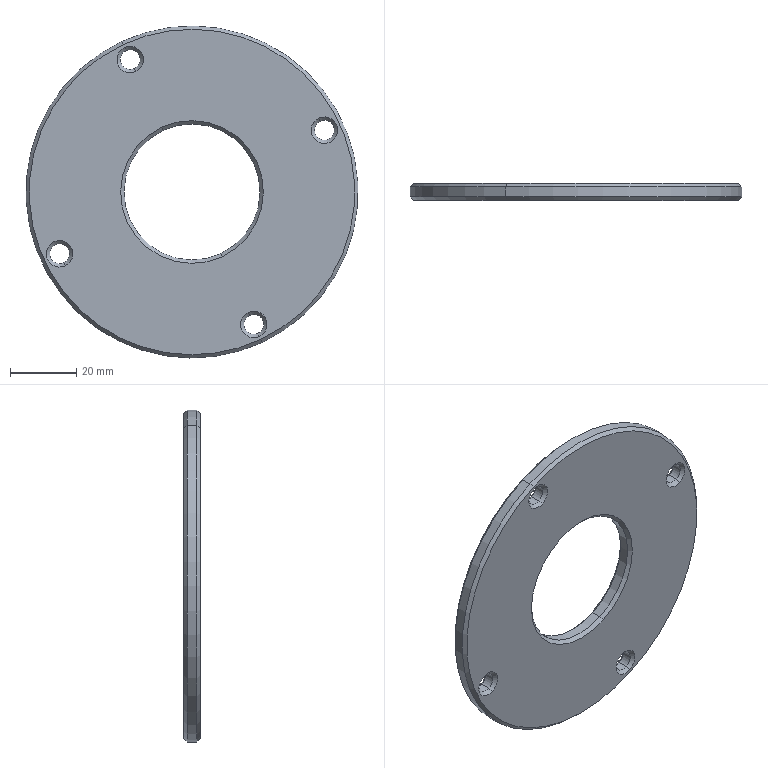Component | SolidWorks | BearingHousingAssembly-1_BearingCoverPlate-1 | 1 solid | 38 faces | box 100 x 5 x 100 mm | volume 31576 mm3 | cone 24 | cylinder 12 | plane 2 | commonest cylinder face diameters 6 x8 41 x2 100 x2 | material Plain Carbon Steel
STEP:
#1=COLOUR_RGB('',0.7922,0.8196,0.9333);
#2=FILL_AREA_STYLE_COLOUR('',#1);
#3=FILL_AREA_STYLE('',(#2));
#4=SURFACE_STYLE_FILL_AREA(#3);
#5=SURFACE_SIDE_STYLE('',(#4));
#6=SURFACE_STYLE_USAGE(.BOTH.,#5);
#7=PRESENTATION_STYLE_ASSIGNMENT((#6));
#8=CARTESIAN_POINT('',(-2.304,9.577,1.441));
#9=VERTEX_POINT('',#8);
#10=CARTESIAN_POINT('',(-2.204,9.577,1.227));
#11=VERTEX_POINT('',#10);
#12=CARTESIAN_POINT('',(-2.254,9.577,1.334));
#13=DIRECTION('',(-0.,-1.,-0.));
#14=DIRECTION('',(0.4226,0.,-0.9063));
#15=AXIS2_PLACEMENT_3D('',#12,#13,#14);
#16=CIRCLE('',#15,0.1181);
#17=EDGE_CURVE('',#9,#11,#16,.T.);
#18=ORIENTED_EDGE('',*,*,#17,.F.);
#19=CARTESIAN_POINT('',(-2.321,9.538,1.476));
#20=VERTEX_POINT('',#19);
#21=CARTESIAN_POINT('',(-2.304,9.577,1.441));
#22=DIRECTION('',(-0.2988,-0.7071,0.6409));
#23=VECTOR('',#22,39.37);
#24=LINE('',#21,#23);
#25=EDGE_CURVE('',#9,#20,#24,.T.);
#26=ORIENTED_EDGE('',*,*,#25,.T.);
#27=CARTESIAN_POINT('',(-2.188,9.538,1.191));
#28=VERTEX_POINT('',#27);
#29=CARTESIAN_POINT('',(-2.254,9.538,1.334));
#30=DIRECTION('',(0.,1.,0.));
#31=DIRECTION('',(0.4226,0.,-0.9063));
#32=AXIS2_PLACEMENT_3D('',#29,#30,#31);
#33=CIRCLE('',#32,0.1575);
#34=EDGE_CURVE('',#28,#20,#33,.T.);
#35=ORIENTED_EDGE('',*,*,#34,.F.);
#36=CARTESIAN_POINT('',(-2.204,9.577,1.227));
#37=DIRECTION('',(0.2988,-0.7071,-0.6409));
#38=VECTOR('',#37,39.37);
#39=LINE('',#36,#38);
#40=EDGE_CURVE('',#11,#28,#39,.T.);
#41=ORIENTED_EDGE('',*,*,#40,.F.);
#42=EDGE_LOOP('',(#18,#26,#35,#41));
#43=FACE_OUTER_BOUND('',#42,.T.);
#44=CARTESIAN_POINT('',(-2.254,9.577,1.334));
#45=DIRECTION('',(-0.,-1.,-0.));
#46=DIRECTION('',(0.4226,0.,-0.9063));
#47=AXIS2_PLACEMENT_3D('',#44,#45,#46);
#48=CONICAL_SURFACE('',#47,0.1181,0.7854);
#49=ADVANCED_FACE('',(#43),#48,.F.);
#50=CARTESIAN_POINT('',(-3.142,9.577,-0.8613));
#51=VERTEX_POINT('',#50);
#52=CARTESIAN_POINT('',(-3.042,9.577,-1.075));
#53=VERTEX_POINT('',#52);
#54=CARTESIAN_POINT('',(-3.092,9.577,-0.9683));
#55=DIRECTION('',(-0.,-1.,-0.));
#56=DIRECTION('',(0.4226,0.,-0.9063));
#57=AXIS2_PLACEMENT_3D('',#54,#55,#56);
#58=CIRCLE('',#57,0.1181);
#59=EDGE_CURVE('',#51,#53,#58,.T.);
#60=ORIENTED_EDGE('',*,*,#59,.F.);
#61=CARTESIAN_POINT('',(-3.159,9.538,-0.8256));
#62=VERTEX_POINT('',#61);
#63=CARTESIAN_POINT('',(-3.142,9.577,-0.8613));
#64=DIRECTION('',(-0.2988,-0.7071,0.6409));
#65=VECTOR('',#64,39.37);
#66=LINE('',#63,#65);
#67=EDGE_CURVE('',#51,#62,#66,.T.);
#68=ORIENTED_EDGE('',*,*,#67,.T.);
#69=CARTESIAN_POINT('',(-3.026,9.538,-1.111));
#70=VERTEX_POINT('',#69);
#71=CARTESIAN_POINT('',(-3.092,9.538,-0.9683));
#72=DIRECTION('',(0.,1.,0.));
#73=DIRECTION('',(0.4226,0.,-0.9063));
#74=AXIS2_PLACEMENT_3D('',#71,#72,#73);
#75=CIRCLE('',#74,0.1575);
#76=EDGE_CURVE('',#70,#62,#75,.T.);
#77=ORIENTED_EDGE('',*,*,#76,.F.);
#78=CARTESIAN_POINT('',(-3.042,9.577,-1.075));
#79=DIRECTION('',(0.2988,-0.7071,-0.6409));
#80=VECTOR('',#79,39.37);
#81=LINE('',#78,#80);
#82=EDGE_CURVE('',#53,#70,#81,.T.);
#83=ORIENTED_EDGE('',*,*,#82,.F.);
#84=EDGE_LOOP('',(#60,#68,#77,#83));
#85=FACE_OUTER_BOUND('',#84,.T.);
#86=CARTESIAN_POINT('',(-3.092,9.577,-0.9683));
#87=DIRECTION('',(-0.,-1.,-0.));
#88=DIRECTION('',(0.4226,0.,-0.9063));
#89=AXIS2_PLACEMENT_3D('',#86,#87,#88);
#90=CONICAL_SURFACE('',#89,0.1181,0.7854);
#91=ADVANCED_FACE('',(#85),#90,.F.);
#92=CARTESIAN_POINT('',(-0.8401,9.577,-1.699));
#93=VERTEX_POINT('',#92);
#94=CARTESIAN_POINT('',(-0.7403,9.577,-1.913));
#95=VERTEX_POINT('',#94);
#96=CARTESIAN_POINT('',(-0.7902,9.577,-1.806));
#97=DIRECTION('',(-0.,-1.,-0.));
#98=DIRECTION('',(0.4226,0.,-0.9063));
#99=AXIS2_PLACEMENT_3D('',#96,#97,#98);
#100=CIRCLE('',#99,0.1181);
#101=EDGE_CURVE('',#93,#95,#100,.T.);
#102=ORIENTED_EDGE('',*,*,#101,.F.);
#103=CARTESIAN_POINT('',(-0.8567,9.538,-1.663));
#104=VERTEX_POINT('',#103);
#105=CARTESIAN_POINT('',(-0.8401,9.577,-1.699));
#106=DIRECTION('',(-0.2988,-0.7071,0.6409));
#107=VECTOR('',#106,39.37);
#108=LINE('',#105,#107);
#109=EDGE_CURVE('',#93,#104,#108,.T.);
#110=ORIENTED_EDGE('',*,*,#109,.T.);
#111=CARTESIAN_POINT('',(-0.7236,9.538,-1.949));
#112=VERTEX_POINT('',#111);
#113=CARTESIAN_POINT('',(-0.7902,9.538,-1.806));
#114=DIRECTION('',(0.,1.,0.));
#115=DIRECTION('',(0.4226,0.,-0.9063));
#116=AXIS2_PLACEMENT_3D('',#113,#114,#115);
#117=CIRCLE('',#116,0.1575);
#118=EDGE_CURVE('',#112,#104,#117,.T.);
#119=ORIENTED_EDGE('',*,*,#118,.F.);
#120=CARTESIAN_POINT('',(-0.7403,9.577,-1.913));
#121=DIRECTION('',(0.2988,-0.7071,-0.6409));
#122=VECTOR('',#121,39.37);
#123=LINE('',#120,#122);
#124=EDGE_CURVE('',#95,#112,#123,.T.);
#125=ORIENTED_EDGE('',*,*,#124,.F.);
#126=EDGE_LOOP('',(#102,#110,#119,#125));
#127=FACE_OUTER_BOUND('',#126,.T.);
#128=CARTESIAN_POINT('',(-0.7902,9.577,-1.806));
#129=DIRECTION('',(-0.,-1.,-0.));
#130=DIRECTION('',(0.4226,0.,-0.9063));
#131=AXIS2_PLACEMENT_3D('',#128,#129,#130);
#132=CONICAL_SURFACE('',#131,0.1181,0.7854);
#133=ADVANCED_FACE('',(#127),#132,.F.);
#134=CARTESIAN_POINT('',(-0.002213,9.577,0.6029));
#135=VERTEX_POINT('',#134);
#136=CARTESIAN_POINT('',(0.09762,9.577,0.3888));
#137=VERTEX_POINT('',#136);
#138=CARTESIAN_POINT('',(0.0477,9.577,0.4959));
#139=DIRECTION('',(-0.,-1.,-0.));
#140=DIRECTION('',(0.4226,0.,-0.9063));
#141=AXIS2_PLACEMENT_3D('',#138,#139,#140);
#142=CIRCLE('',#141,0.1181);
#143=EDGE_CURVE('',#135,#137,#142,.T.);
#144=ORIENTED_EDGE('',*,*,#143,.F.);
#145=CARTESIAN_POINT('',(-0.01885,9.538,0.6386));
#146=VERTEX_POINT('',#145);
#147=CARTESIAN_POINT('',(-0.002213,9.577,0.6029));
#148=DIRECTION('',(-0.2988,-0.7071,0.6409));
#149=VECTOR('',#148,39.37);
#150=LINE('',#147,#149);
#151=EDGE_CURVE('',#135,#146,#150,.T.);
#152=ORIENTED_EDGE('',*,*,#151,.T.);
#153=CARTESIAN_POINT('',(0.1143,9.538,0.3531));
#154=VERTEX_POINT('',#153);
#155=CARTESIAN_POINT('',(0.0477,9.538,0.4959));
#156=DIRECTION('',(0.,1.,0.));
#157=DIRECTION('',(0.4226,0.,-0.9063));
#158=AXIS2_PLACEMENT_3D('',#155,#156,#157);
#159=CIRCLE('',#158,0.1575);
#160=EDGE_CURVE('',#154,#146,#159,.T.);
#161=ORIENTED_EDGE('',*,*,#160,.F.);
#162=CARTESIAN_POINT('',(0.09762,9.577,0.3888));
#163=DIRECTION('',(0.2988,-0.7071,-0.6409));
#164=VECTOR('',#163,39.37);
#165=LINE('',#162,#164);
#166=EDGE_CURVE('',#137,#154,#165,.T.);
#167=ORIENTED_EDGE('',*,*,#166,.F.);
#168=EDGE_LOOP('',(#144,#152,#161,#167));
#169=FACE_OUTER_BOUND('',#168,.T.);
#170=CARTESIAN_POINT('',(0.0477,9.577,0.4959));
#171=DIRECTION('',(-0.,-1.,-0.));
#172=DIRECTION('',(0.4226,0.,-0.9063));
#173=AXIS2_PLACEMENT_3D('',#170,#171,#172);
#174=CONICAL_SURFACE('',#173,0.1181,0.7854);
#175=ADVANCED_FACE('',(#169),#174,.F.);
#176=CARTESIAN_POINT('',(-0.707,9.538,-1.985));
#177=VERTEX_POINT('',#176);
#178=CARTESIAN_POINT('',(-2.338,9.538,1.512));
#179=VERTEX_POINT('',#178);
#180=CARTESIAN_POINT('',(-1.522,9.538,-0.2362));
#181=DIRECTION('',(-0.,-1.,-0.));
#182=DIRECTION('',(0.4226,0.,-0.9063));
#183=AXIS2_PLACEMENT_3D('',#180,#181,#182);
#184=CIRCLE('',#183,1.929);
#185=EDGE_CURVE('',#177,#179,#184,.T.);
#186=ORIENTED_EDGE('',*,*,#185,.F.);
#187=CARTESIAN_POINT('',(-0.6904,9.577,-2.02));
#188=VERTEX_POINT('',#187);
#189=CARTESIAN_POINT('',(-0.707,9.538,-1.985));
#190=DIRECTION('',(0.2988,0.7071,-0.6409));
#191=VECTOR('',#190,39.37);
#192=LINE('',#189,#191);
#193=EDGE_CURVE('',#177,#188,#192,.T.);
#194=ORIENTED_EDGE('',*,*,#193,.T.);
#195=CARTESIAN_POINT('',(-2.354,9.577,1.548));
#196=VERTEX_POINT('',#195);
#197=CARTESIAN_POINT('',(-1.522,9.577,-0.2362));
#198=DIRECTION('',(0.,1.,0.));
#199=DIRECTION('',(0.4226,0.,-0.9063));
#200=AXIS2_PLACEMENT_3D('',#197,#198,#199);
#201=CIRCLE('',#200,1.969);
#202=EDGE_CURVE('',#196,#188,#201,.T.);
#203=ORIENTED_EDGE('',*,*,#202,.F.);
#204=CARTESIAN_POINT('',(-2.338,9.538,1.512));
#205=DIRECTION('',(-0.2988,0.7071,0.6409));
#206=VECTOR('',#205,39.37);
#207=LINE('',#204,#206);
#208=EDGE_CURVE('',#179,#196,#207,.T.);
#209=ORIENTED_EDGE('',*,*,#208,.F.);
#210=EDGE_LOOP('',(#186,#194,#203,#209));
#211=FACE_OUTER_BOUND('',#210,.T.);
#212=CARTESIAN_POINT('',(-1.522,9.538,-0.2362));
#213=DIRECTION('',(0.,1.,0.));
#214=DIRECTION('',(-0.4226,0.,0.9063));
#215=AXIS2_PLACEMENT_3D('',#212,#213,#214);
#216=CONICAL_SURFACE('',#215,1.929,0.7854);
#217=ADVANCED_FACE('',(#211),#216,.T.);
#218=CARTESIAN_POINT('',(-1.863,9.577,0.4952));
#219=VERTEX_POINT('',#218);
#220=CARTESIAN_POINT('',(-1.181,9.577,-0.9677));
#221=VERTEX_POINT('',#220);
#222=CARTESIAN_POINT('',(-1.522,9.577,-0.2362));
#223=DIRECTION('',(-0.,-1.,-0.));
#224=DIRECTION('',(0.4226,0.,-0.9063));
#225=AXIS2_PLACEMENT_3D('',#222,#223,#224);
#226=CIRCLE('',#225,0.8071);
#227=EDGE_CURVE('',#219,#221,#226,.T.);
#228=ORIENTED_EDGE('',*,*,#227,.F.);
#229=CARTESIAN_POINT('',(-1.88,9.538,0.5309));
#230=VERTEX_POINT('',#229);
#231=CARTESIAN_POINT('',(-1.863,9.577,0.4952));
#232=DIRECTION('',(-0.2988,-0.7071,0.6409));
#233=VECTOR('',#232,39.37);
#234=LINE('',#231,#233);
#235=EDGE_CURVE('',#219,#230,#234,.T.);
#236=ORIENTED_EDGE('',*,*,#235,.T.);
#237=CARTESIAN_POINT('',(-1.165,9.538,-1.003));
#238=VERTEX_POINT('',#237);
#239=CARTESIAN_POINT('',(-1.522,9.538,-0.2362));
#240=DIRECTION('',(0.,1.,0.));
#241=DIRECTION('',(0.4226,0.,-0.9063));
#242=AXIS2_PLACEMENT_3D('',#239,#240,#241);
#243=CIRCLE('',#242,0.8465);
#244=EDGE_CURVE('',#238,#230,#243,.T.);
#245=ORIENTED_EDGE('',*,*,#244,.F.);
#246=CARTESIAN_POINT('',(-1.181,9.577,-0.9677));
#247=DIRECTION('',(0.2988,-0.7071,-0.6409));
#248=VECTOR('',#247,39.37);
#249=LINE('',#246,#248);
#250=EDGE_CURVE('',#221,#238,#249,.T.);
#251=ORIENTED_EDGE('',*,*,#250,.F.);
#252=EDGE_LOOP('',(#228,#236,#245,#251));
#253=FACE_OUTER_BOUND('',#252,.T.);
#254=CARTESIAN_POINT('',(-1.522,9.577,-0.2362));
#255=DIRECTION('',(-0.,-1.,-0.));
#256=DIRECTION('',(0.4226,0.,-0.9063));
#257=AXIS2_PLACEMENT_3D('',#254,#255,#256);
#258=CONICAL_SURFACE('',#257,0.8071,0.7854);
#259=ADVANCED_FACE('',(#253),#258,.F.);
#260=CARTESIAN_POINT('',(-2.204,9.695,1.227));
#261=VERTEX_POINT('',#260);
#262=CARTESIAN_POINT('',(-2.304,9.695,1.441));
#263=VERTEX_POINT('',#262);
#264=CARTESIAN_POINT('',(-2.254,9.695,1.334));
#265=DIRECTION('',(0.,1.,0.));
#266=DIRECTION('',(0.4226,0.,-0.9063));
#267=AXIS2_PLACEMENT_3D('',#264,#265,#266);
#268=CIRCLE('',#267,0.1181);
#269=EDGE_CURVE('',#261,#263,#268,.T.);
#270=ORIENTED_EDGE('',*,*,#269,.F.);
#271=CARTESIAN_POINT('',(-2.188,9.735,1.191));
#272=VERTEX_POINT('',#271);
#273=CARTESIAN_POINT('',(-2.188,9.735,1.191));
#274=DIRECTION('',(0.2988,0.7071,-0.6409));
#275=VECTOR('',#274,39.37);
#276=LINE('',#273,#275);
#277=EDGE_CURVE('',#261,#272,#276,.T.);
#278=ORIENTED_EDGE('',*,*,#277,.T.);
#279=CARTESIAN_POINT('',(-2.321,9.735,1.476));
#280=VERTEX_POINT('',#279);
#281=CARTESIAN_POINT('',(-2.254,9.735,1.334));
#282=DIRECTION('',(-0.,-1.,-0.));
#283=DIRECTION('',(0.4226,0.,-0.9063));
#284=AXIS2_PLACEMENT_3D('',#281,#282,#283);
#285=CIRCLE('',#284,0.1575);
#286=EDGE_CURVE('',#280,#272,#285,.T.);
#287=ORIENTED_EDGE('',*,*,#286,.F.);
#288=CARTESIAN_POINT('',(-2.321,9.735,1.476));
#289=DIRECTION('',(-0.2988,0.7071,0.6409));
#290=VECTOR('',#289,39.37);
#291=LINE('',#288,#290);
#292=EDGE_CURVE('',#263,#280,#291,.T.);
#293=ORIENTED_EDGE('',*,*,#292,.F.);
#294=EDGE_LOOP('',(#270,#278,#287,#293));
#295=FACE_OUTER_BOUND('',#294,.T.);
#296=CARTESIAN_POINT('',(-2.254,9.735,1.334));
#297=DIRECTION('',(0.,1.,0.));
#298=DIRECTION('',(-0.4226,0.,0.9063));
#299=AXIS2_PLACEMENT_3D('',#296,#297,#298);
#300=CONICAL_SURFACE('',#299,0.1575,0.7854);
#301=ADVANCED_FACE('',(#295),#300,.F.);
#302=CARTESIAN_POINT('',(-3.042,9.695,-1.075));
#303=VERTEX_POINT('',#302);
#304=CARTESIAN_POINT('',(-3.142,9.695,-0.8613));
#305=VERTEX_POINT('',#304);
#306=CARTESIAN_POINT('',(-3.092,9.695,-0.9683));
#307=DIRECTION('',(0.,1.,0.));
#308=DIRECTION('',(0.4226,0.,-0.9063));
#309=AXIS2_PLACEMENT_3D('',#306,#307,#308);
#310=CIRCLE('',#309,0.1181);
#311=EDGE_CURVE('',#303,#305,#310,.T.);
#312=ORIENTED_EDGE('',*,*,#311,.F.);
#313=CARTESIAN_POINT('',(-3.026,9.735,-1.111));
#314=VERTEX_POINT('',#313);
#315=CARTESIAN_POINT('',(-3.026,9.735,-1.111));
#316=DIRECTION('',(0.2988,0.7071,-0.6409));
#317=VECTOR('',#316,39.37);
#318=LINE('',#315,#317);
#319=EDGE_CURVE('',#303,#314,#318,.T.);
#320=ORIENTED_EDGE('',*,*,#319,.T.);
#321=CARTESIAN_POINT('',(-3.159,9.735,-0.8256));
#322=VERTEX_POINT('',#321);
#323=CARTESIAN_POINT('',(-3.092,9.735,-0.9683));
#324=DIRECTION('',(-0.,-1.,-0.));
#325=DIRECTION('',(0.4226,0.,-0.9063));
#326=AXIS2_PLACEMENT_3D('',#323,#324,#325);
#327=CIRCLE('',#326,0.1575);
#328=EDGE_CURVE('',#322,#314,#327,.T.);
#329=ORIENTED_EDGE('',*,*,#328,.F.);
#330=CARTESIAN_POINT('',(-3.159,9.735,-0.8256));
#331=DIRECTION('',(-0.2988,0.7071,0.6409));
#332=VECTOR('',#331,39.37);
#333=LINE('',#330,#332);
#334=EDGE_CURVE('',#305,#322,#333,.T.);
#335=ORIENTED_EDGE('',*,*,#334,.F.);
#336=EDGE_LOOP('',(#312,#320,#329,#335));
#337=FACE_OUTER_BOUND('',#336,.T.);
#338=CARTESIAN_POINT('',(-3.092,9.735,-0.9683));
#339=DIRECTION('',(0.,1.,0.));
#340=DIRECTION('',(-0.4226,0.,0.9063));
#341=AXIS2_PLACEMENT_3D('',#338,#339,#340);
#342=CONICAL_SURFACE('',#341,0.1575,0.7854);
#343=ADVANCED_FACE('',(#337),#342,.F.);
#344=CARTESIAN_POINT('',(-0.7403,9.695,-1.913));
#345=VERTEX_POINT('',#344);
#346=CARTESIAN_POINT('',(-0.8401,9.695,-1.699));
#347=VERTEX_POINT('',#346);
#348=CARTESIAN_POINT('',(-0.7902,9.695,-1.806));
#349=DIRECTION('',(0.,1.,0.));
#350=DIRECTION('',(0.4226,0.,-0.9063));
#351=AXIS2_PLACEMENT_3D('',#348,#349,#350);
#352=CIRCLE('',#351,0.1181);
#353=EDGE_CURVE('',#345,#347,#352,.T.);
#354=ORIENTED_EDGE('',*,*,#353,.F.);
#355=CARTESIAN_POINT('',(-0.7236,9.735,-1.949));
#356=VERTEX_POINT('',#355);
#357=CARTESIAN_POINT('',(-0.7236,9.735,-1.949));
#358=DIRECTION('',(0.2988,0.7071,-0.6409));
#359=VECTOR('',#358,39.37);
#360=LINE('',#357,#359);
#361=EDGE_CURVE('',#345,#356,#360,.T.);
#362=ORIENTED_EDGE('',*,*,#361,.T.);
#363=CARTESIAN_POINT('',(-0.8567,9.735,-1.663));
#364=VERTEX_POINT('',#363);
#365=CARTESIAN_POINT('',(-0.7902,9.735,-1.806));
#366=DIRECTION('',(-0.,-1.,-0.));
#367=DIRECTION('',(0.4226,0.,-0.9063));
#368=AXIS2_PLACEMENT_3D('',#365,#366,#367);
#369=CIRCLE('',#368,0.1575);
#370=EDGE_CURVE('',#364,#356,#369,.T.);
#371=ORIENTED_EDGE('',*,*,#370,.F.);
#372=CARTESIAN_POINT('',(-0.8567,9.735,-1.663));
#373=DIRECTION('',(-0.2988,0.7071,0.6409));
#374=VECTOR('',#373,39.37);
#375=LINE('',#372,#374);
#376=EDGE_CURVE('',#347,#364,#375,.T.);
#377=ORIENTED_EDGE('',*,*,#376,.F.);
#378=EDGE_LOOP('',(#354,#362,#371,#377));
#379=FACE_OUTER_BOUND('',#378,.T.);
#380=CARTESIAN_POINT('',(-0.7902,9.735,-1.806));
#381=DIRECTION('',(0.,1.,0.));
#382=DIRECTION('',(-0.4226,0.,0.9063));
#383=AXIS2_PLACEMENT_3D('',#380,#381,#382);
#384=CONICAL_SURFACE('',#383,0.1575,0.7854);
#385=ADVANCED_FACE('',(#379),#384,.F.);
#386=CARTESIAN_POINT('',(0.09762,9.695,0.3888));
#387=VERTEX_POINT('',#386);
#388=CARTESIAN_POINT('',(-0.002213,9.695,0.6029));
#389=VERTEX_POINT('',#388);
#390=CARTESIAN_POINT('',(0.0477,9.695,0.4959));
#391=DIRECTION('',(0.,1.,0.));
#392=DIRECTION('',(0.4226,0.,-0.9063));
#393=AXIS2_PLACEMENT_3D('',#390,#391,#392);
#394=CIRCLE('',#393,0.1181);
#395=EDGE_CURVE('',#387,#389,#394,.T.);
#396=ORIENTED_EDGE('',*,*,#395,.F.);
#397=CARTESIAN_POINT('',(0.1143,9.735,0.3531));
#398=VERTEX_POINT('',#397);
#399=CARTESIAN_POINT('',(0.1143,9.735,0.3531));
#400=DIRECTION('',(0.2988,0.7071,-0.6409));
#401=VECTOR('',#400,39.37);
#402=LINE('',#399,#401);
#403=EDGE_CURVE('',#387,#398,#402,.T.);
#404=ORIENTED_EDGE('',*,*,#403,.T.);
#405=CARTESIAN_POINT('',(-0.01885,9.735,0.6386));
#406=VERTEX_POINT('',#405);
#407=CARTESIAN_POINT('',(0.0477,9.735,0.4959));
#408=DIRECTION('',(-0.,-1.,-0.));
#409=DIRECTION('',(0.4226,0.,-0.9063));
#410=AXIS2_PLACEMENT_3D('',#407,#408,#409);
#411=CIRCLE('',#410,0.1575);
#412=EDGE_CURVE('',#406,#398,#411,.T.);
#413=ORIENTED_EDGE('',*,*,#412,.F.);
#414=CARTESIAN_POINT('',(-0.01885,9.735,0.6386));
#415=DIRECTION('',(-0.2988,0.7071,0.6409));
#416=VECTOR('',#415,39.37);
#417=LINE('',#414,#416);
#418=EDGE_CURVE('',#389,#406,#417,.T.);
#419=ORIENTED_EDGE('',*,*,#418,.F.);
#420=EDGE_LOOP('',(#396,#404,#413,#419));
#421=FACE_OUTER_BOUND('',#420,.T.);
#422=CARTESIAN_POINT('',(0.0477,9.735,0.4959));
#423=DIRECTION('',(0.,1.,0.));
#424=DIRECTION('',(-0.4226,0.,0.9063));
#425=AXIS2_PLACEMENT_3D('',#422,#423,#424);
#426=CONICAL_SURFACE('',#425,0.1575,0.7854);
#427=ADVANCED_FACE('',(#421),#426,.F.);
#428=CARTESIAN_POINT('',(-2.338,9.735,1.512));
#429=VERTEX_POINT('',#428);
#430=CARTESIAN_POINT('',(-0.707,9.735,-1.985));
#431=VERTEX_POINT('',#430);
#432=CARTESIAN_POINT('',(-1.522,9.735,-0.2362));
#433=DIRECTION('',(0.,1.,0.));
#434=DIRECTION('',(0.4226,0.,-0.9063));
#435=AXIS2_PLACEMENT_3D('',#432,#433,#434);
#436=CIRCLE('',#435,1.929);
#437=EDGE_CURVE('',#429,#431,#436,.T.);
#438=ORIENTED_EDGE('',*,*,#437,.F.);
#439=CARTESIAN_POINT('',(-2.354,9.695,1.548));
#440=VERTEX_POINT('',#439);
#441=CARTESIAN_POINT('',(-2.354,9.695,1.548));
#442=DIRECTION('',(-0.2988,-0.7071,0.6409));
#443=VECTOR('',#442,39.37);
#444=LINE('',#441,#443);
#445=EDGE_CURVE('',#429,#440,#444,.T.);
#446=ORIENTED_EDGE('',*,*,#445,.T.);
#447=CARTESIAN_POINT('',(-0.6904,9.695,-2.02));
#448=VERTEX_POINT('',#447);
#449=CARTESIAN_POINT('',(-1.522,9.695,-0.2362));
#450=DIRECTION('',(-0.,-1.,-0.));
#451=DIRECTION('',(0.4226,0.,-0.9063));
#452=AXIS2_PLACEMENT_3D('',#449,#450,#451);
#453=CIRCLE('',#452,1.969);
#454=EDGE_CURVE('',#448,#440,#453,.T.);
#455=ORIENTED_EDGE('',*,*,#454,.F.);
#456=CARTESIAN_POINT('',(-0.6904,9.695,-2.02));
#457=DIRECTION('',(0.2988,-0.7071,-0.6409));
#458=VECTOR('',#457,39.37);
#459=LINE('',#456,#458);
#460=EDGE_CURVE('',#431,#448,#459,.T.);
#461=ORIENTED_EDGE('',*,*,#460,.F.);
#462=EDGE_LOOP('',(#438,#446,#455,#461));
#463=FACE_OUTER_BOUND('',#462,.T.);
#464=CARTESIAN_POINT('',(-1.522,9.695,-0.2362));
#465=DIRECTION('',(-0.,-1.,-0.));
#466=DIRECTION('',(0.4226,0.,-0.9063));
#467=AXIS2_PLACEMENT_3D('',#464,#465,#466);
#468=CONICAL_SURFACE('',#467,1.969,0.7854);
#469=ADVANCED_FACE('',(#463),#468,.T.);
#470=CARTESIAN_POINT('',(-1.181,9.695,-0.9677));
#471=VERTEX_POINT('',#470);
#472=CARTESIAN_POINT('',(-1.863,9.695,0.4952));
#473=VERTEX_POINT('',#472);
#474=CARTESIAN_POINT('',(-1.522,9.695,-0.2362));
#475=DIRECTION('',(0.,1.,0.));
#476=DIRECTION('',(0.4226,0.,-0.9063));
#477=AXIS2_PLACEMENT_3D('',#474,#475,#476);
#478=CIRCLE('',#477,0.8071);
#479=EDGE_CURVE('',#471,#473,#478,.T.);
#480=ORIENTED_EDGE('',*,*,#479,.F.);
#481=CARTESIAN_POINT('',(-1.165,9.735,-1.003));
#482=VERTEX_POINT('',#481);
#483=CARTESIAN_POINT('',(-1.165,9.735,-1.003));
#484=DIRECTION('',(0.2988,0.7071,-0.6409));
#485=VECTOR('',#484,39.37);
#486=LINE('',#483,#485);
#487=EDGE_CURVE('',#471,#482,#486,.T.);
#488=ORIENTED_EDGE('',*,*,#487,.T.);
#489=CARTESIAN_POINT('',(-1.88,9.735,0.5309));
#490=VERTEX_POINT('',#489);
#491=CARTESIAN_POINT('',(-1.522,9.735,-0.2362));
#492=DIRECTION('',(-0.,-1.,-0.));
#493=DIRECTION('',(0.4226,0.,-0.9063));
#494=AXIS2_PLACEMENT_3D('',#491,#492,#493);
#495=CIRCLE('',#494,0.8465);
#496=EDGE_CURVE('',#490,#482,#495,.T.);
#497=ORIENTED_EDGE('',*,*,#496,.F.);
#498=CARTESIAN_POINT('',(-1.88,9.735,0.5309));
#499=DIRECTION('',(-0.2988,0.7071,0.6409));
#500=VECTOR('',#499,39.37);
#501=LINE('',#498,#500);
#502=EDGE_CURVE('',#473,#490,#501,.T.);
#503=ORIENTED_EDGE('',*,*,#502,.F.);
#504=EDGE_LOOP('',(#480,#488,#497,#503));
#505=FACE_OUTER_BOUND('',#504,.T.);
#506=CARTESIAN_POINT('',(-1.522,9.735,-0.2362));
#507=DIRECTION('',(0.,1.,0.));
#508=DIRECTION('',(-0.4226,0.,0.9063));
#509=AXIS2_PLACEMENT_3D('',#506,#507,#508);
#510=CONICAL_SURFACE('',#509,0.8465,0.7854);
#511=ADVANCED_FACE('',(#505),#510,.F.);
#512=ORIENTED_EDGE('',*,*,#269,.T.);
#513=CARTESIAN_POINT('',(-2.304,9.735,1.441));
#514=DIRECTION('',(-0.,-1.,-0.));
#515=VECTOR('',#514,39.37);
#516=LINE('',#513,#515);
#517=EDGE_CURVE('',#263,#9,#516,.T.);
#518=ORIENTED_EDGE('',*,*,#517,.T.);
#519=ORIENTED_EDGE('',*,*,#17,.T.);
#520=CARTESIAN_POINT('',(-2.204,9.735,1.227));
#521=DIRECTION('',(-0.,-1.,-0.));
#522=VECTOR('',#521,39.37);
#523=LINE('',#520,#522);
#524=EDGE_CURVE('',#261,#11,#523,.T.);
#525=ORIENTED_EDGE('',*,*,#524,.F.);
#526=EDGE_LOOP('',(#512,#518,#519,#525));
#527=FACE_OUTER_BOUND('',#526,.T.);
#528=CARTESIAN_POINT('',(-2.254,9.735,1.334));
#529=DIRECTION('',(-0.,-1.,-0.));
#530=DIRECTION('',(0.4226,0.,-0.9063));
#531=AXIS2_PLACEMENT_3D('',#528,#529,#530);
#532=CYLINDRICAL_SURFACE('',#531,0.1181);
#533=ADVANCED_FACE('',(#527),#532,.F.);
#534=ORIENTED_EDGE('',*,*,#311,.T.);
#535=CARTESIAN_POINT('',(-3.142,9.735,-0.8613));
#536=DIRECTION('',(-0.,-1.,-0.));
#537=VECTOR('',#536,39.37);
#538=LINE('',#535,#537);
#539=EDGE_CURVE('',#305,#51,#538,.T.);
#540=ORIENTED_EDGE('',*,*,#539,.T.);
#541=ORIENTED_EDGE('',*,*,#59,.T.);
#542=CARTESIAN_POINT('',(-3.042,9.735,-1.075));
#543=DIRECTION('',(-0.,-1.,-0.));
#544=VECTOR('',#543,39.37);
#545=LINE('',#542,#544);
#546=EDGE_CURVE('',#303,#53,#545,.T.);
#547=ORIENTED_EDGE('',*,*,#546,.F.);
#548=EDGE_LOOP('',(#534,#540,#541,#547));
#549=FACE_OUTER_BOUND('',#548,.T.);
#550=CARTESIAN_POINT('',(-3.092,9.735,-0.9683));
#551=DIRECTION('',(-0.,-1.,-0.));
#552=DIRECTION('',(0.4226,0.,-0.9063));
#553=AXIS2_PLACEMENT_3D('',#550,#551,#552);
#554=CYLINDRICAL_SURFACE('',#553,0.1181);
#555=ADVANCED_FACE('',(#549),#554,.F.);
#556=ORIENTED_EDGE('',*,*,#353,.T.);
#557=CARTESIAN_POINT('',(-0.8401,9.735,-1.699));
#558=DIRECTION('',(-0.,-1.,-0.));
#559=VECTOR('',#558,39.37);
#560=LINE('',#557,#559);
#561=EDGE_CURVE('',#347,#93,#560,.T.);
#562=ORIENTED_EDGE('',*,*,#561,.T.);
#563=ORIENTED_EDGE('',*,*,#101,.T.);
#564=CARTESIAN_POINT('',(-0.7403,9.735,-1.913));
#565=DIRECTION('',(-0.,-1.,-0.));
#566=VECTOR('',#565,39.37);
#567=LINE('',#564,#566);
#568=EDGE_CURVE('',#345,#95,#567,.T.);
#569=ORIENTED_EDGE('',*,*,#568,.F.);
#570=EDGE_LOOP('',(#556,#562,#563,#569));
#571=FACE_OUTER_BOUND('',#570,.T.);
#572=CARTESIAN_POINT('',(-0.7902,9.735,-1.806));
#573=DIRECTION('',(-0.,-1.,-0.));
#574=DIRECTION('',(0.4226,0.,-0.9063));
#575=AXIS2_PLACEMENT_3D('',#572,#573,#574);
#576=CYLINDRICAL_SURFACE('',#575,0.1181);
#577=ADVANCED_FACE('',(#571),#576,.F.);
#578=ORIENTED_EDGE('',*,*,#395,.T.);
#579=CARTESIAN_POINT('',(-0.002213,9.735,0.6029));
#580=DIRECTION('',(-0.,-1.,-0.));
#581=VECTOR('',#580,39.37);
#582=LINE('',#579,#581);
#583=EDGE_CURVE('',#389,#135,#582,.T.);
#584=ORIENTED_EDGE('',*,*,#583,.T.);
#585=ORIENTED_EDGE('',*,*,#143,.T.);
#586=CARTESIAN_POINT('',(0.09762,9.735,0.3888));
#587=DIRECTION('',(-0.,-1.,-0.));
#588=VECTOR('',#587,39.37);
#589=LINE('',#586,#588);
#590=EDGE_CURVE('',#387,#137,#589,.T.);
#591=ORIENTED_EDGE('',*,*,#590,.F.);
#592=EDGE_LOOP('',(#578,#584,#585,#591));
#593=FACE_OUTER_BOUND('',#592,.T.);
#594=CARTESIAN_POINT('',(0.0477,9.735,0.4959));
#595=DIRECTION('',(-0.,-1.,-0.));
#596=DIRECTION('',(0.4226,0.,-0.9063));
#597=AXIS2_PLACEMENT_3D('',#594,#595,#596);
#598=CYLINDRICAL_SURFACE('',#597,0.1181);
#599=ADVANCED_FACE('',(#593),#598,.F.);
#600=ORIENTED_EDGE('',*,*,#227,.T.);
#601=CARTESIAN_POINT('',(-1.181,9.538,-0.9677));
#602=DIRECTION('',(0.,1.,0.));
#603=VECTOR('',#602,39.37);
#604=LINE('',#601,#603);
#605=EDGE_CURVE('',#221,#471,#604,.T.);
#606=ORIENTED_EDGE('',*,*,#605,.T.);
#607=ORIENTED_EDGE('',*,*,#479,.T.);
#608=CARTESIAN_POINT('',(-1.863,9.538,0.4952));
#609=DIRECTION('',(0.,1.,0.));
#610=VECTOR('',#609,39.37);
#611=LINE('',#608,#610);
#612=EDGE_CURVE('',#219,#473,#611,.T.);
#613=ORIENTED_EDGE('',*,*,#612,.F.);
#614=EDGE_LOOP('',(#600,#606,#607,#613));
#615=FACE_OUTER_BOUND('',#614,.T.);
#616=CARTESIAN_POINT('',(-1.522,9.538,-0.2362));
#617=DIRECTION('',(0.,1.,0.));
#618=DIRECTION('',(-0.4226,0.,0.9063));
#619=AXIS2_PLACEMENT_3D('',#616,#617,#618);
#620=CYLINDRICAL_SURFACE('',#619,0.8071);
#621=ADVANCED_FACE('',(#615),#620,.F.);
#622=ORIENTED_EDGE('',*,*,#202,.T.);
#623=CARTESIAN_POINT('',(-0.6904,9.538,-2.02));
#624=DIRECTION('',(0.,1.,0.));
#625=VECTOR('',#624,39.37);
#626=LINE('',#623,#625);
#627=EDGE_CURVE('',#188,#448,#626,.T.);
#628=ORIENTED_EDGE('',*,*,#627,.T.);
#629=ORIENTED_EDGE('',*,*,#454,.T.);
#630=CARTESIAN_POINT('',(-2.354,9.538,1.548));
#631=DIRECTION('',(0.,1.,0.));
#632=VECTOR('',#631,39.37);
#633=LINE('',#630,#632);
#634=EDGE_CURVE('',#196,#440,#633,.T.);
#635=ORIENTED_EDGE('',*,*,#634,.F.);
#636=EDGE_LOOP('',(#622,#628,#629,#635));
#637=FACE_OUTER_BOUND('',#636,.T.);
#638=CARTESIAN_POINT('',(-1.522,9.538,-0.2362));
#639=DIRECTION('',(0.,1.,0.));
#640=DIRECTION('',(-0.4226,0.,0.9063));
#641=AXIS2_PLACEMENT_3D('',#638,#639,#640);
#642=CYLINDRICAL_SURFACE('',#641,1.969);
#643=ADVANCED_FACE('',(#637),#642,.T.);
#644=ORIENTED_EDGE('',*,*,#244,.T.);
#645=CARTESIAN_POINT('',(-1.522,9.538,-0.2362));
#646=DIRECTION('',(0.,1.,0.));
#647=DIRECTION('',(0.4226,0.,-0.9063));
#648=AXIS2_PLACEMENT_3D('',#645,#646,#647);
#649=CIRCLE('',#648,0.8465);
#650=EDGE_CURVE('',#230,#238,#649,.T.);
#651=ORIENTED_EDGE('',*,*,#650,.T.);
#652=EDGE_LOOP('',(#644,#651));
#653=FACE_BOUND('',#652,.T.);
#654=CARTESIAN_POINT('',(-1.522,9.538,-0.2362));
#655=DIRECTION('',(-0.,-1.,-0.));
#656=DIRECTION('',(0.4226,0.,-0.9063));
#657=AXIS2_PLACEMENT_3D('',#654,#655,#656);
#658=CIRCLE('',#657,1.929);
#659=EDGE_CURVE('',#179,#177,#658,.T.);
#660=ORIENTED_EDGE('',*,*,#659,.T.);
#661=ORIENTED_EDGE('',*,*,#185,.T.);
#662=EDGE_LOOP('',(#660,#661));
#663=FACE_OUTER_BOUND('',#662,.T.);
#664=ORIENTED_EDGE('',*,*,#160,.T.);
#665=CARTESIAN_POINT('',(0.0477,9.538,0.4959));
#666=DIRECTION('',(0.,1.,0.));
#667=DIRECTION('',(0.4226,0.,-0.9063));
#668=AXIS2_PLACEMENT_3D('',#665,#666,#667);
#669=CIRCLE('',#668,0.1575);
#670=EDGE_CURVE('',#146,#154,#669,.T.);
#671=ORIENTED_EDGE('',*,*,#670,.T.);
#672=EDGE_LOOP('',(#664,#671));
#673=FACE_BOUND('',#672,.T.);
#674=ORIENTED_EDGE('',*,*,#118,.T.);
#675=CARTESIAN_POINT('',(-0.7902,9.538,-1.806));
#676=DIRECTION('',(0.,1.,0.));
#677=DIRECTION('',(0.4226,0.,-0.9063));
#678=AXIS2_PLACEMENT_3D('',#675,#676,#677);
#679=CIRCLE('',#678,0.1575);
#680=EDGE_CURVE('',#104,#112,#679,.T.);
#681=ORIENTED_EDGE('',*,*,#680,.T.);
#682=EDGE_LOOP('',(#674,#681));
#683=FACE_BOUND('',#682,.T.);
#684=ORIENTED_EDGE('',*,*,#76,.T.);
#685=CARTESIAN_POINT('',(-3.092,9.538,-0.9683));
#686=DIRECTION('',(0.,1.,0.));
#687=DIRECTION('',(0.4226,0.,-0.9063));
#688=AXIS2_PLACEMENT_3D('',#685,#686,#687);
#689=CIRCLE('',#688,0.1575);
#690=EDGE_CURVE('',#62,#70,#689,.T.);
#691=ORIENTED_EDGE('',*,*,#690,.T.);
#692=EDGE_LOOP('',(#684,#691));
#693=FACE_BOUND('',#692,.T.);
#694=ORIENTED_EDGE('',*,*,#34,.T.);
#695=CARTESIAN_POINT('',(-2.254,9.538,1.334));
#696=DIRECTION('',(0.,1.,0.));
#697=DIRECTION('',(0.4226,0.,-0.9063));
#698=AXIS2_PLACEMENT_3D('',#695,#696,#697);
#699=CIRCLE('',#698,0.1575);
#700=EDGE_CURVE('',#20,#28,#699,.T.);
#701=ORIENTED_EDGE('',*,*,#700,.T.);
#702=EDGE_LOOP('',(#694,#701));
#703=FACE_BOUND('',#702,.T.);
#704=CARTESIAN_POINT('',(-1.522,9.538,-0.2362));
#705=DIRECTION('',(-0.,-1.,-0.));
#706=DIRECTION('',(0.4226,-0.,-0.9063));
#707=AXIS2_PLACEMENT_3D('',#704,#705,#706);
#708=PLANE('',#707);
#709=ADVANCED_FACE('',(#653,#663,#673,#683,#693,#703),#708,.T.);
#710=ORIENTED_EDGE('',*,*,#496,.T.);
#711=CARTESIAN_POINT('',(-1.522,9.735,-0.2362));
#712=DIRECTION('',(-0.,-1.,-0.));
#713=DIRECTION('',(0.4226,0.,-0.9063));
#714=AXIS2_PLACEMENT_3D('',#711,#712,#713);
#715=CIRCLE('',#714,0.8465);
#716=EDGE_CURVE('',#482,#490,#715,.T.);
#717=ORIENTED_EDGE('',*,*,#716,.T.);
#718=EDGE_LOOP('',(#710,#717));
#719=FACE_BOUND('',#718,.T.);
#720=CARTESIAN_POINT('',(-1.522,9.735,-0.2362));
#721=DIRECTION('',(0.,1.,0.));
#722=DIRECTION('',(0.4226,0.,-0.9063));
#723=AXIS2_PLACEMENT_3D('',#720,#721,#722);
#724=CIRCLE('',#723,1.929);
#725=EDGE_CURVE('',#431,#429,#724,.T.);
#726=ORIENTED_EDGE('',*,*,#725,.T.);
#727=ORIENTED_EDGE('',*,*,#437,.T.);
#728=EDGE_LOOP('',(#726,#727));
#729=FACE_OUTER_BOUND('',#728,.T.);
#730=ORIENTED_EDGE('',*,*,#412,.T.);
#731=CARTESIAN_POINT('',(0.0477,9.735,0.4959));
#732=DIRECTION('',(-0.,-1.,-0.));
#733=DIRECTION('',(0.4226,0.,-0.9063));
#734=AXIS2_PLACEMENT_3D('',#731,#732,#733);
#735=CIRCLE('',#734,0.1575);
#736=EDGE_CURVE('',#398,#406,#735,.T.);
#737=ORIENTED_EDGE('',*,*,#736,.T.);
#738=EDGE_LOOP('',(#730,#737));
#739=FACE_BOUND('',#738,.T.);
#740=ORIENTED_EDGE('',*,*,#370,.T.);
#741=CARTESIAN_POINT('',(-0.7902,9.735,-1.806));
#742=DIRECTION('',(-0.,-1.,-0.));
#743=DIRECTION('',(0.4226,0.,-0.9063));
#744=AXIS2_PLACEMENT_3D('',#741,#742,#743);
#745=CIRCLE('',#744,0.1575);
#746=EDGE_CURVE('',#356,#364,#745,.T.);
#747=ORIENTED_EDGE('',*,*,#746,.T.);
#748=EDGE_LOOP('',(#740,#747));
#749=FACE_BOUND('',#748,.T.);
#750=ORIENTED_EDGE('',*,*,#328,.T.);
#751=CARTESIAN_POINT('',(-3.092,9.735,-0.9683));
#752=DIRECTION('',(-0.,-1.,-0.));
#753=DIRECTION('',(0.4226,0.,-0.9063));
#754=AXIS2_PLACEMENT_3D('',#751,#752,#753);
#755=CIRCLE('',#754,0.1575);
#756=EDGE_CURVE('',#314,#322,#755,.T.);
#757=ORIENTED_EDGE('',*,*,#756,.T.);
#758=EDGE_LOOP('',(#750,#757));
#759=FACE_BOUND('',#758,.T.);
#760=ORIENTED_EDGE('',*,*,#286,.T.);
#761=CARTESIAN_POINT('',(-2.254,9.735,1.334));
#762=DIRECTION('',(-0.,-1.,-0.));
#763=DIRECTION('',(0.4226,0.,-0.9063));
#764=AXIS2_PLACEMENT_3D('',#761,#762,#763);
#765=CIRCLE('',#764,0.1575);
#766=EDGE_CURVE('',#272,#280,#765,.T.);
#767=ORIENTED_EDGE('',*,*,#766,.T.);
#768=EDGE_LOOP('',(#760,#767));
#769=FACE_BOUND('',#768,.T.);
#770=CARTESIAN_POINT('',(-1.522,9.735,-0.2362));
#771=DIRECTION('',(-0.,-1.,-0.));
#772=DIRECTION('',(0.4226,-0.,-0.9063));
#773=AXIS2_PLACEMENT_3D('',#770,#771,#772);
#774=PLANE('',#773);
#775=ADVANCED_FACE('',(#719,#729,#739,#749,#759,#769),#774,.F.);
#776=ORIENTED_EDGE('',*,*,#627,.F.);
#777=CARTESIAN_POINT('',(-1.522,9.577,-0.2362));
#778=DIRECTION('',(0.,1.,0.));
#779=DIRECTION('',(0.4226,0.,-0.9063));
#780=AXIS2_PLACEMENT_3D('',#777,#778,#779);
#781=CIRCLE('',#780,1.969);
#782=EDGE_CURVE('',#188,#196,#781,.T.);
#783=ORIENTED_EDGE('',*,*,#782,.T.);
#784=ORIENTED_EDGE('',*,*,#634,.T.);
#785=CARTESIAN_POINT('',(-1.522,9.695,-0.2362));
#786=DIRECTION('',(-0.,-1.,-0.));
#787=DIRECTION('',(0.4226,0.,-0.9063));
#788=AXIS2_PLACEMENT_3D('',#785,#786,#787);
#789=CIRCLE('',#788,1.969);
#790=EDGE_CURVE('',#440,#448,#789,.T.);
#791=ORIENTED_EDGE('',*,*,#790,.T.);
#792=EDGE_LOOP('',(#776,#783,#784,#791));
#793=FACE_OUTER_BOUND('',#792,.T.);
#794=CARTESIAN_POINT('',(-1.522,9.538,-0.2362));
#795=DIRECTION('',(0.,1.,0.));
#796=DIRECTION('',(-0.4226,0.,0.9063));
#797=AXIS2_PLACEMENT_3D('',#794,#795,#796);
#798=CYLINDRICAL_SURFACE('',#797,1.969);
#799=ADVANCED_FACE('',(#793),#798,.T.);
#800=ORIENTED_EDGE('',*,*,#605,.F.);
#801=CARTESIAN_POINT('',(-1.522,9.577,-0.2362));
#802=DIRECTION('',(-0.,-1.,-0.));
#803=DIRECTION('',(0.4226,0.,-0.9063));
#804=AXIS2_PLACEMENT_3D('',#801,#802,#803);
#805=CIRCLE('',#804,0.8071);
#806=EDGE_CURVE('',#221,#219,#805,.T.);
#807=ORIENTED_EDGE('',*,*,#806,.T.);
#808=ORIENTED_EDGE('',*,*,#612,.T.);
#809=CARTESIAN_POINT('',(-1.522,9.695,-0.2362));
#810=DIRECTION('',(0.,1.,0.));
#811=DIRECTION('',(0.4226,0.,-0.9063));
#812=AXIS2_PLACEMENT_3D('',#809,#810,#811);
#813=CIRCLE('',#812,0.8071);
#814=EDGE_CURVE('',#473,#471,#813,.T.);
#815=ORIENTED_EDGE('',*,*,#814,.T.);
#816=EDGE_LOOP('',(#800,#807,#808,#815));
#817=FACE_OUTER_BOUND('',#816,.T.);
#818=CARTESIAN_POINT('',(-1.522,9.538,-0.2362));
#819=DIRECTION('',(0.,1.,0.));
#820=DIRECTION('',(-0.4226,0.,0.9063));
#821=AXIS2_PLACEMENT_3D('',#818,#819,#820);
#822=CYLINDRICAL_SURFACE('',#821,0.8071);
#823=ADVANCED_FACE('',(#817),#822,.F.);
#824=ORIENTED_EDGE('',*,*,#583,.F.);
#825=CARTESIAN_POINT('',(0.0477,9.695,0.4959));
#826=DIRECTION('',(0.,1.,0.));
#827=DIRECTION('',(0.4226,0.,-0.9063));
#828=AXIS2_PLACEMENT_3D('',#825,#826,#827);
#829=CIRCLE('',#828,0.1181);
#830=EDGE_CURVE('',#389,#387,#829,.T.);
#831=ORIENTED_EDGE('',*,*,#830,.T.);
#832=ORIENTED_EDGE('',*,*,#590,.T.);
#833=CARTESIAN_POINT('',(0.0477,9.577,0.4959));
#834=DIRECTION('',(-0.,-1.,-0.));
#835=DIRECTION('',(0.4226,0.,-0.9063));
#836=AXIS2_PLACEMENT_3D('',#833,#834,#835);
#837=CIRCLE('',#836,0.1181);
#838=EDGE_CURVE('',#137,#135,#837,.T.);
#839=ORIENTED_EDGE('',*,*,#838,.T.);
#840=EDGE_LOOP('',(#824,#831,#832,#839));
#841=FACE_OUTER_BOUND('',#840,.T.);
#842=CARTESIAN_POINT('',(0.0477,9.735,0.4959));
#843=DIRECTION('',(-0.,-1.,-0.));
#844=DIRECTION('',(0.4226,0.,-0.9063));
#845=AXIS2_PLACEMENT_3D('',#842,#843,#844);
#846=CYLINDRICAL_SURFACE('',#845,0.1181);
#847=ADVANCED_FACE('',(#841),#846,.F.);
#848=ORIENTED_EDGE('',*,*,#561,.F.);
#849=CARTESIAN_POINT('',(-0.7902,9.695,-1.806));
#850=DIRECTION('',(0.,1.,0.));
#851=DIRECTION('',(0.4226,0.,-0.9063));
#852=AXIS2_PLACEMENT_3D('',#849,#850,#851);
#853=CIRCLE('',#852,0.1181);
#854=EDGE_CURVE('',#347,#345,#853,.T.);
#855=ORIENTED_EDGE('',*,*,#854,.T.);
#856=ORIENTED_EDGE('',*,*,#568,.T.);
#857=CARTESIAN_POINT('',(-0.7902,9.577,-1.806));
#858=DIRECTION('',(-0.,-1.,-0.));
#859=DIRECTION('',(0.4226,0.,-0.9063));
#860=AXIS2_PLACEMENT_3D('',#857,#858,#859);
#861=CIRCLE('',#860,0.1181);
#862=EDGE_CURVE('',#95,#93,#861,.T.);
#863=ORIENTED_EDGE('',*,*,#862,.T.);
#864=EDGE_LOOP('',(#848,#855,#856,#863));
#865=FACE_OUTER_BOUND('',#864,.T.);
#866=CARTESIAN_POINT('',(-0.7902,9.735,-1.806));
#867=DIRECTION('',(-0.,-1.,-0.));
#868=DIRECTION('',(0.4226,0.,-0.9063));
#869=AXIS2_PLACEMENT_3D('',#866,#867,#868);
#870=CYLINDRICAL_SURFACE('',#869,0.1181);
#871=ADVANCED_FACE('',(#865),#870,.F.);
#872=ORIENTED_EDGE('',*,*,#539,.F.);
#873=CARTESIAN_POINT('',(-3.092,9.695,-0.9683));
#874=DIRECTION('',(0.,1.,0.));
#875=DIRECTION('',(0.4226,0.,-0.9063));
#876=AXIS2_PLACEMENT_3D('',#873,#874,#875);
#877=CIRCLE('',#876,0.1181);
#878=EDGE_CURVE('',#305,#303,#877,.T.);
#879=ORIENTED_EDGE('',*,*,#878,.T.);
#880=ORIENTED_EDGE('',*,*,#546,.T.);
#881=CARTESIAN_POINT('',(-3.092,9.577,-0.9683));
#882=DIRECTION('',(-0.,-1.,-0.));
#883=DIRECTION('',(0.4226,0.,-0.9063));
#884=AXIS2_PLACEMENT_3D('',#881,#882,#883);
#885=CIRCLE('',#884,0.1181);
#886=EDGE_CURVE('',#53,#51,#885,.T.);
#887=ORIENTED_EDGE('',*,*,#886,.T.);
#888=EDGE_LOOP('',(#872,#879,#880,#887));
#889=FACE_OUTER_BOUND('',#888,.T.);
#890=CARTESIAN_POINT('',(-3.092,9.735,-0.9683));
#891=DIRECTION('',(-0.,-1.,-0.));
#892=DIRECTION('',(0.4226,0.,-0.9063));
#893=AXIS2_PLACEMENT_3D('',#890,#891,#892);
#894=CYLINDRICAL_SURFACE('',#893,0.1181);
#895=ADVANCED_FACE('',(#889),#894,.F.);
#896=ORIENTED_EDGE('',*,*,#517,.F.);
#897=CARTESIAN_POINT('',(-2.254,9.695,1.334));
#898=DIRECTION('',(0.,1.,0.));
#899=DIRECTION('',(0.4226,0.,-0.9063));
#900=AXIS2_PLACEMENT_3D('',#897,#898,#899);
#901=CIRCLE('',#900,0.1181);
#902=EDGE_CURVE('',#263,#261,#901,.T.);
#903=ORIENTED_EDGE('',*,*,#902,.T.);
#904=ORIENTED_EDGE('',*,*,#524,.T.);
#905=CARTESIAN_POINT('',(-2.254,9.577,1.334));
#906=DIRECTION('',(-0.,-1.,-0.));
#907=DIRECTION('',(0.4226,0.,-0.9063));
#908=AXIS2_PLACEMENT_3D('',#905,#906,#907);
#909=CIRCLE('',#908,0.1181);
#910=EDGE_CURVE('',#11,#9,#909,.T.);
#911=ORIENTED_EDGE('',*,*,#910,.T.);
#912=EDGE_LOOP('',(#896,#903,#904,#911));
#913=FACE_OUTER_BOUND('',#912,.T.);
#914=CARTESIAN_POINT('',(-2.254,9.735,1.334));
#915=DIRECTION('',(-0.,-1.,-0.));
#916=DIRECTION('',(0.4226,0.,-0.9063));
#917=AXIS2_PLACEMENT_3D('',#914,#915,#916);
#918=CYLINDRICAL_SURFACE('',#917,0.1181);
#919=ADVANCED_FACE('',(#913),#918,.F.);
#920=ORIENTED_EDGE('',*,*,#487,.F.);
#921=ORIENTED_EDGE('',*,*,#814,.F.);
#922=ORIENTED_EDGE('',*,*,#502,.T.);
#923=ORIENTED_EDGE('',*,*,#716,.F.);
#924=EDGE_LOOP('',(#920,#921,#922,#923));
#925=FACE_OUTER_BOUND('',#924,.T.);
#926=CARTESIAN_POINT('',(-1.522,9.735,-0.2362));
#927=DIRECTION('',(0.,1.,0.));
#928=DIRECTION('',(-0.4226,0.,0.9063));
#929=AXIS2_PLACEMENT_3D('',#926,#927,#928);
#930=CONICAL_SURFACE('',#929,0.8465,0.7854);
#931=ADVANCED_FACE('',(#925),#930,.F.);
#932=ORIENTED_EDGE('',*,*,#445,.F.);
#933=ORIENTED_EDGE('',*,*,#725,.F.);
#934=ORIENTED_EDGE('',*,*,#460,.T.);
#935=ORIENTED_EDGE('',*,*,#790,.F.);
#936=EDGE_LOOP('',(#932,#933,#934,#935));
#937=FACE_OUTER_BOUND('',#936,.T.);
#938=CARTESIAN_POINT('',(-1.522,9.695,-0.2362));
#939=DIRECTION('',(-0.,-1.,-0.));
#940=DIRECTION('',(0.4226,0.,-0.9063));
#941=AXIS2_PLACEMENT_3D('',#938,#939,#940);
#942=CONICAL_SURFACE('',#941,1.969,0.7854);
#943=ADVANCED_FACE('',(#937),#942,.T.);
#944=ORIENTED_EDGE('',*,*,#403,.F.);
#945=ORIENTED_EDGE('',*,*,#830,.F.);
#946=ORIENTED_EDGE('',*,*,#418,.T.);
#947=ORIENTED_EDGE('',*,*,#736,.F.);
#948=EDGE_LOOP('',(#944,#945,#946,#947));
#949=FACE_OUTER_BOUND('',#948,.T.);
#950=CARTESIAN_POINT('',(0.0477,9.735,0.4959));
#951=DIRECTION('',(0.,1.,0.));
#952=DIRECTION('',(-0.4226,0.,0.9063));
#953=AXIS2_PLACEMENT_3D('',#950,#951,#952);
#954=CONICAL_SURFACE('',#953,0.1575,0.7854);
#955=ADVANCED_FACE('',(#949),#954,.F.);
#956=ORIENTED_EDGE('',*,*,#361,.F.);
#957=ORIENTED_EDGE('',*,*,#854,.F.);
#958=ORIENTED_EDGE('',*,*,#376,.T.);
#959=ORIENTED_EDGE('',*,*,#746,.F.);
#960=EDGE_LOOP('',(#956,#957,#958,#959));
#961=FACE_OUTER_BOUND('',#960,.T.);
#962=CARTESIAN_POINT('',(-0.7902,9.735,-1.806));
#963=DIRECTION('',(0.,1.,0.));
#964=DIRECTION('',(-0.4226,0.,0.9063));
#965=AXIS2_PLACEMENT_3D('',#962,#963,#964);
#966=CONICAL_SURFACE('',#965,0.1575,0.7854);
#967=ADVANCED_FACE('',(#961),#966,.F.);
#968=ORIENTED_EDGE('',*,*,#319,.F.);
#969=ORIENTED_EDGE('',*,*,#878,.F.);
#970=ORIENTED_EDGE('',*,*,#334,.T.);
#971=ORIENTED_EDGE('',*,*,#756,.F.);
#972=EDGE_LOOP('',(#968,#969,#970,#971));
#973=FACE_OUTER_BOUND('',#972,.T.);
#974=CARTESIAN_POINT('',(-3.092,9.735,-0.9683));
#975=DIRECTION('',(0.,1.,0.));
#976=DIRECTION('',(-0.4226,0.,0.9063));
#977=AXIS2_PLACEMENT_3D('',#974,#975,#976);
#978=CONICAL_SURFACE('',#977,0.1575,0.7854);
#979=ADVANCED_FACE('',(#973),#978,.F.);
#980=ORIENTED_EDGE('',*,*,#277,.F.);
#981=ORIENTED_EDGE('',*,*,#902,.F.);
#982=ORIENTED_EDGE('',*,*,#292,.T.);
#983=ORIENTED_EDGE('',*,*,#766,.F.);
#984=EDGE_LOOP('',(#980,#981,#982,#983));
#985=FACE_OUTER_BOUND('',#984,.T.);
#986=CARTESIAN_POINT('',(-2.254,9.735,1.334));
#987=DIRECTION('',(0.,1.,0.));
#988=DIRECTION('',(-0.4226,0.,0.9063));
#989=AXIS2_PLACEMENT_3D('',#986,#987,#988);
#990=CONICAL_SURFACE('',#989,0.1575,0.7854);
#991=ADVANCED_FACE('',(#985),#990,.F.);
#992=ORIENTED_EDGE('',*,*,#235,.F.);
#993=ORIENTED_EDGE('',*,*,#806,.F.);
#994=ORIENTED_EDGE('',*,*,#250,.T.);
#995=ORIENTED_EDGE('',*,*,#650,.F.);
#996=EDGE_LOOP('',(#992,#993,#994,#995));
#997=FACE_OUTER_BOUND('',#996,.T.);
#998=CARTESIAN_POINT('',(-1.522,9.577,-0.2362));
#999=DIRECTION('',(-0.,-1.,-0.));
#1000=DIRECTION('',(0.4226,0.,-0.9063));
#1001=AXIS2_PLACEMENT_3D('',#998,#999,#1000);
#1002=CONICAL_SURFACE('',#1001,0.8071,0.7854);
#1003=ADVANCED_FACE('',(#997),#1002,.F.);
#1004=ORIENTED_EDGE('',*,*,#193,.F.);
#1005=ORIENTED_EDGE('',*,*,#659,.F.);
#1006=ORIENTED_EDGE('',*,*,#208,.T.);
#1007=ORIENTED_EDGE('',*,*,#782,.F.);
#1008=EDGE_LOOP('',(#1004,#1005,#1006,#1007));
#1009=FACE_OUTER_BOUND('',#1008,.T.);
#1010=CARTESIAN_POINT('',(-1.522,9.538,-0.2362));
#1011=DIRECTION('',(0.,1.,0.));
#1012=DIRECTION('',(-0.4226,0.,0.9063));
#1013=AXIS2_PLACEMENT_3D('',#1010,#1011,#1012);
#1014=CONICAL_SURFACE('',#1013,1.929,0.7854);
#1015=ADVANCED_FACE('',(#1009),#1014,.T.);
#1016=ORIENTED_EDGE('',*,*,#151,.F.);
#1017=ORIENTED_EDGE('',*,*,#838,.F.);
#1018=ORIENTED_EDGE('',*,*,#166,.T.);
#1019=ORIENTED_EDGE('',*,*,#670,.F.);
#1020=EDGE_LOOP('',(#1016,#1017,#1018,#1019));
#1021=FACE_OUTER_BOUND('',#1020,.T.);
#1022=CARTESIAN_POINT('',(0.0477,9.577,0.4959));
#1023=DIRECTION('',(-0.,-1.,-0.));
#1024=DIRECTION('',(0.4226,0.,-0.9063));
#1025=AXIS2_PLACEMENT_3D('',#1022,#1023,#1024);
#1026=CONICAL_SURFACE('',#1025,0.1181,0.7854);
#1027=ADVANCED_FACE('',(#1021),#1026,.F.);
#1028=ORIENTED_EDGE('',*,*,#109,.F.);
#1029=ORIENTED_EDGE('',*,*,#862,.F.);
#1030=ORIENTED_EDGE('',*,*,#124,.T.);
#1031=ORIENTED_EDGE('',*,*,#680,.F.);
#1032=EDGE_LOOP('',(#1028,#1029,#1030,#1031));
#1033=FACE_OUTER_BOUND('',#1032,.T.);
#1034=CARTESIAN_POINT('',(-0.7902,9.577,-1.806));
#1035=DIRECTION('',(-0.,-1.,-0.));
#1036=DIRECTION('',(0.4226,0.,-0.9063));
#1037=AXIS2_PLACEMENT_3D('',#1034,#1035,#1036);
#1038=CONICAL_SURFACE('',#1037,0.1181,0.7854);
#1039=ADVANCED_FACE('',(#1033),#1038,.F.);
#1040=ORIENTED_EDGE('',*,*,#67,.F.);
#1041=ORIENTED_EDGE('',*,*,#886,.F.);
#1042=ORIENTED_EDGE('',*,*,#82,.T.);
#1043=ORIENTED_EDGE('',*,*,#690,.F.);
#1044=EDGE_LOOP('',(#1040,#1041,#1042,#1043));
#1045=FACE_OUTER_BOUND('',#1044,.T.);
#1046=CARTESIAN_POINT('',(-3.092,9.577,-0.9683));
#1047=DIRECTION('',(-0.,-1.,-0.));
#1048=DIRECTION('',(0.4226,0.,-0.9063));
#1049=AXIS2_PLACEMENT_3D('',#1046,#1047,#1048);
#1050=CONICAL_SURFACE('',#1049,0.1181,0.7854);
#1051=ADVANCED_FACE('',(#1045),#1050,.F.);
#1052=ORIENTED_EDGE('',*,*,#25,.F.);
#1053=ORIENTED_EDGE('',*,*,#910,.F.);
#1054=ORIENTED_EDGE('',*,*,#40,.T.);
#1055=ORIENTED_EDGE('',*,*,#700,.F.);
#1056=EDGE_LOOP('',(#1052,#1053,#1054,#1055));
#1057=FACE_OUTER_BOUND('',#1056,.T.);
#1058=CARTESIAN_POINT('',(-2.254,9.577,1.334));
#1059=DIRECTION('',(-0.,-1.,-0.));
#1060=DIRECTION('',(0.4226,0.,-0.9063));
#1061=AXIS2_PLACEMENT_3D('',#1058,#1059,#1060);
#1062=CONICAL_SURFACE('',#1061,0.1181,0.7854);
#1063=ADVANCED_FACE('',(#1057),#1062,.F.);
#1064=CLOSED_SHELL('',(#49,#91,#133,#175,#217,#259,#301,#343,#385,#427,#469,#511,#533,#555,#577,#599,#621,#643,#709,#775,#799,#823,#847,#871,#895,#919,#931,#943,#955,#967,#979,#991,#1003,#1015,#1027,#1039,#1051,#1063));
#1065=MANIFOLD_SOLID_BREP('',#1064);
#1066=STYLED_ITEM('',(#7),#1065);
#1067=PRESENTATION_LAYER_ASSIGNMENT('','',(#1066));
#1068=(LENGTH_UNIT()NAMED_UNIT(*)SI_UNIT($,.METRE.));
#1069=LENGTH_MEASURE_WITH_UNIT(LENGTH_MEASURE(0.0254),#1068);
#1070=DIMENSIONAL_EXPONENTS(1.,0.,0.,0.,0.,0.,0.);
#1071=(CONVERSION_BASED_UNIT('',#1069)LENGTH_UNIT()NAMED_UNIT(#1070));
#1072=UNCERTAINTY_MEASURE_WITH_UNIT(LENGTH_MEASURE(0.00001),#1071,'','');
#1073=(NAMED_UNIT(*)PLANE_ANGLE_UNIT()SI_UNIT($,.RADIAN.));
#1074=(NAMED_UNIT(*)SI_UNIT($,.STERADIAN.)SOLID_ANGLE_UNIT());
#1075=(GEOMETRIC_REPRESENTATION_CONTEXT(3)GLOBAL_UNCERTAINTY_ASSIGNED_CONTEXT((#1072))GLOBAL_UNIT_ASSIGNED_CONTEXT((#1071,#1073,#1074))REPRESENTATION_CONTEXT('',''));
#1076=MECHANICAL_DESIGN_GEOMETRIC_PRESENTATION_REPRESENTATION('',(#1066),#1075);
#1077=CARTESIAN_POINT('',(0.,0.,0.));
#1078=DIRECTION('',(0.,0.,1.));
#1079=DIRECTION('',(1.,0.,0.));
#1080=AXIS2_PLACEMENT_3D('',#1077,#1078,#1079);
#1081=(LENGTH_UNIT()NAMED_UNIT(*)SI_UNIT($,.METRE.));
#1082=LENGTH_MEASURE_WITH_UNIT(LENGTH_MEASURE(0.0254),#1081);
#1083=DIMENSIONAL_EXPONENTS(1.,0.,0.,0.,0.,0.,0.);
#1084=(CONVERSION_BASED_UNIT('',#1082)LENGTH_UNIT()NAMED_UNIT(#1083));
#1085=UNCERTAINTY_MEASURE_WITH_UNIT(LENGTH_MEASURE(0.00001),#1084,'','');
#1086=(NAMED_UNIT(*)PLANE_ANGLE_UNIT()SI_UNIT($,.RADIAN.));
#1087=(NAMED_UNIT(*)SI_UNIT($,.STERADIAN.)SOLID_ANGLE_UNIT());
#1088=(GEOMETRIC_REPRESENTATION_CONTEXT(3)GLOBAL_UNCERTAINTY_ASSIGNED_CONTEXT((#1085))GLOBAL_UNIT_ASSIGNED_CONTEXT((#1084,#1086,#1087))REPRESENTATION_CONTEXT('',''));
#1089=ADVANCED_BREP_SHAPE_REPRESENTATION('',(#1065,#1080),#1088);